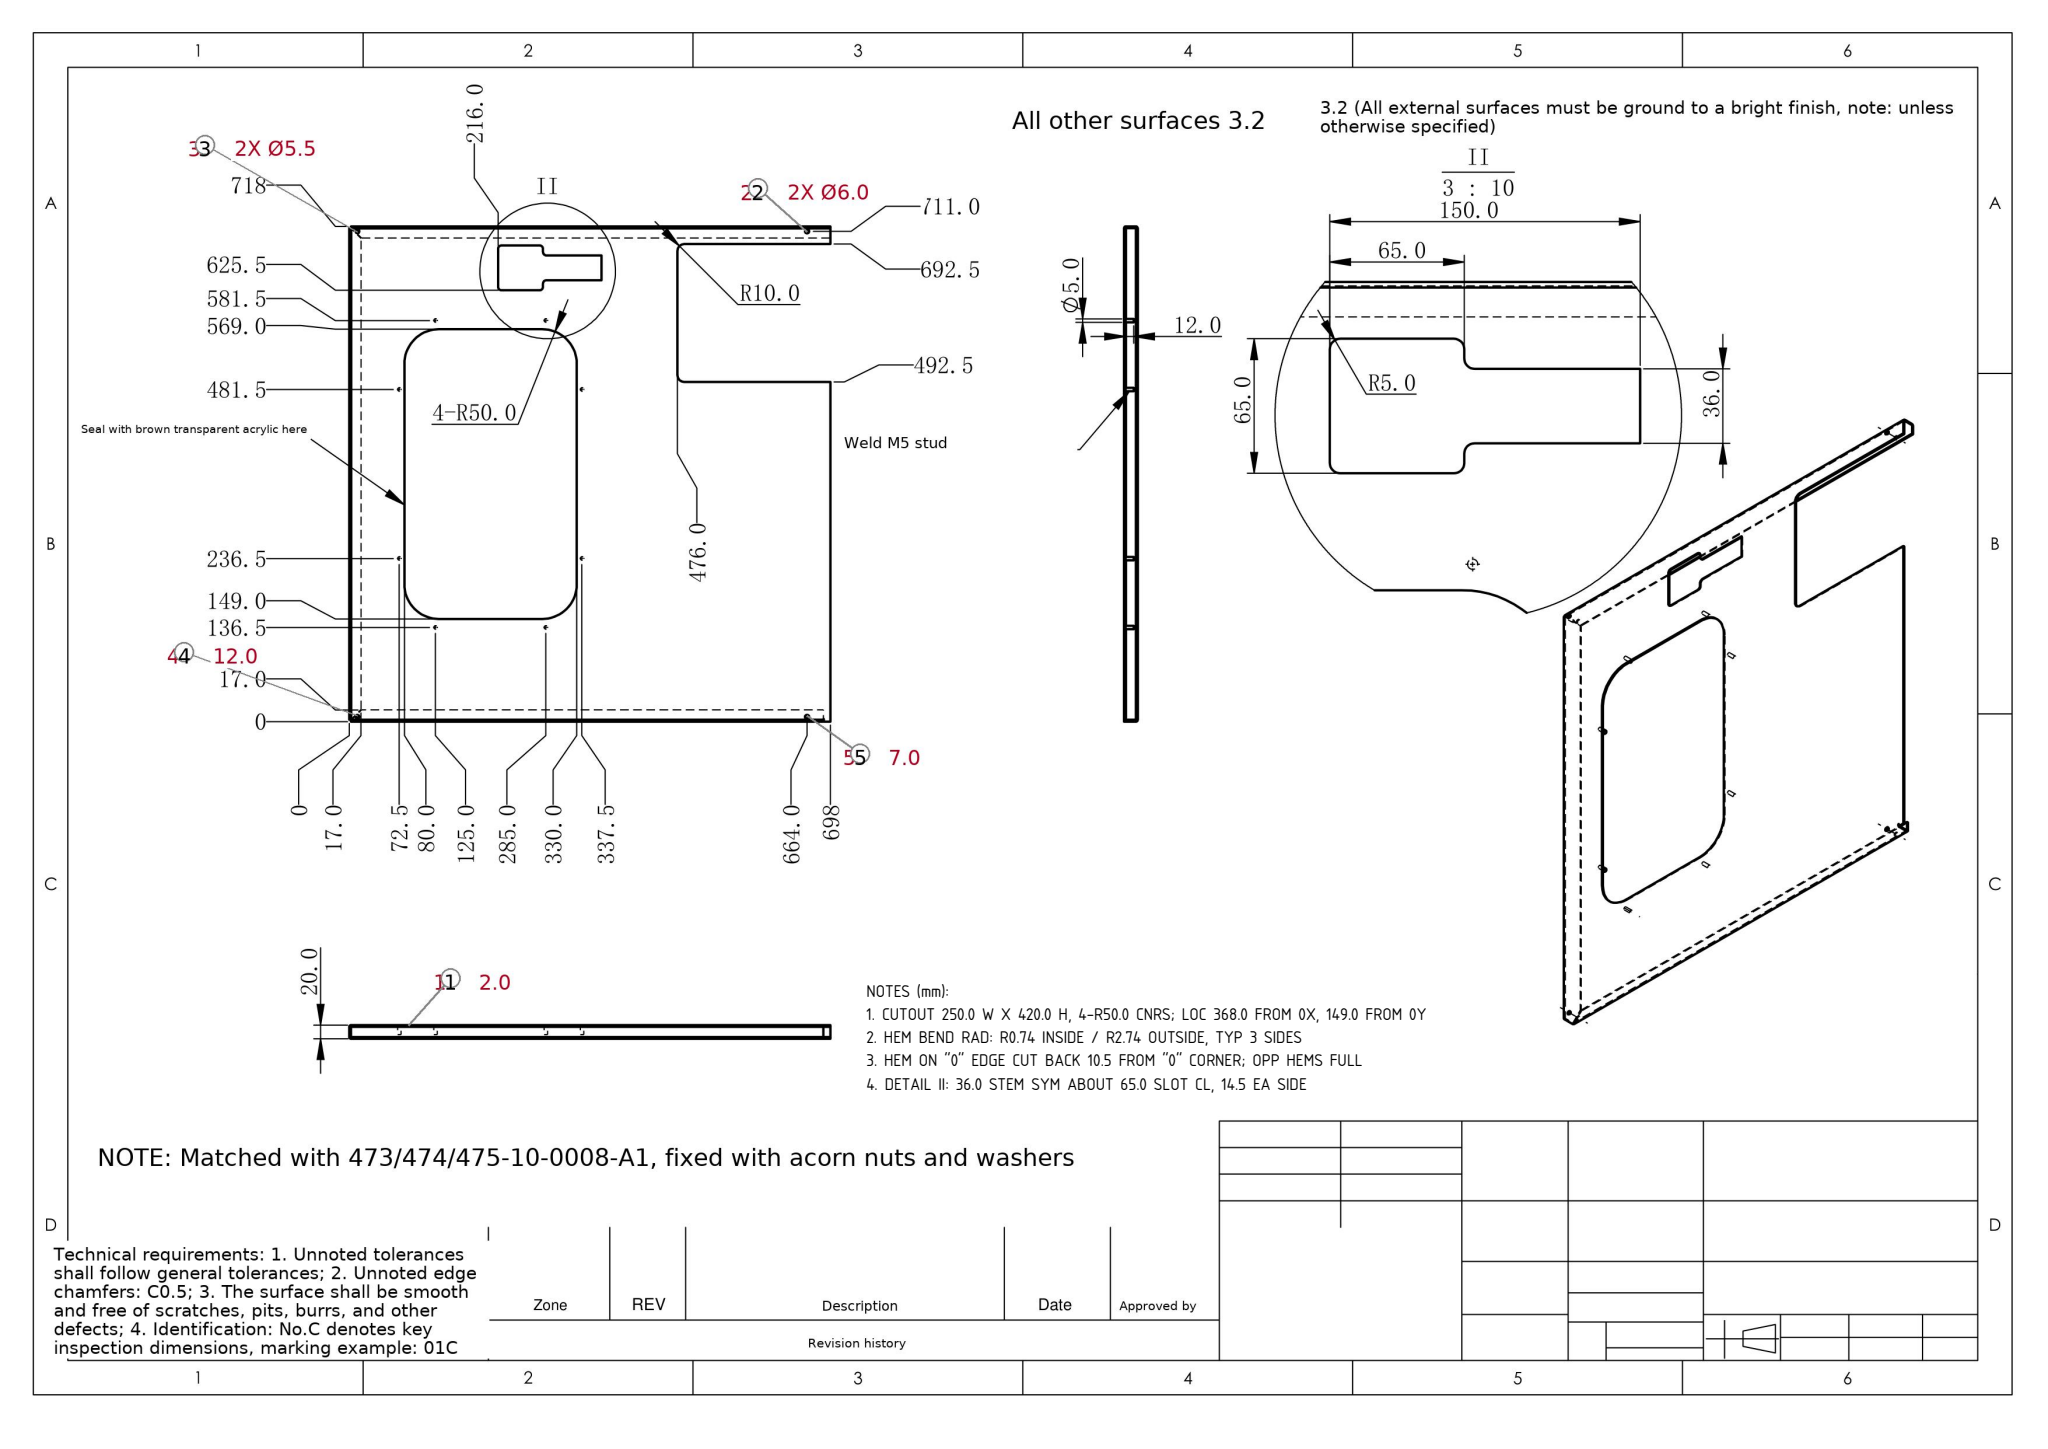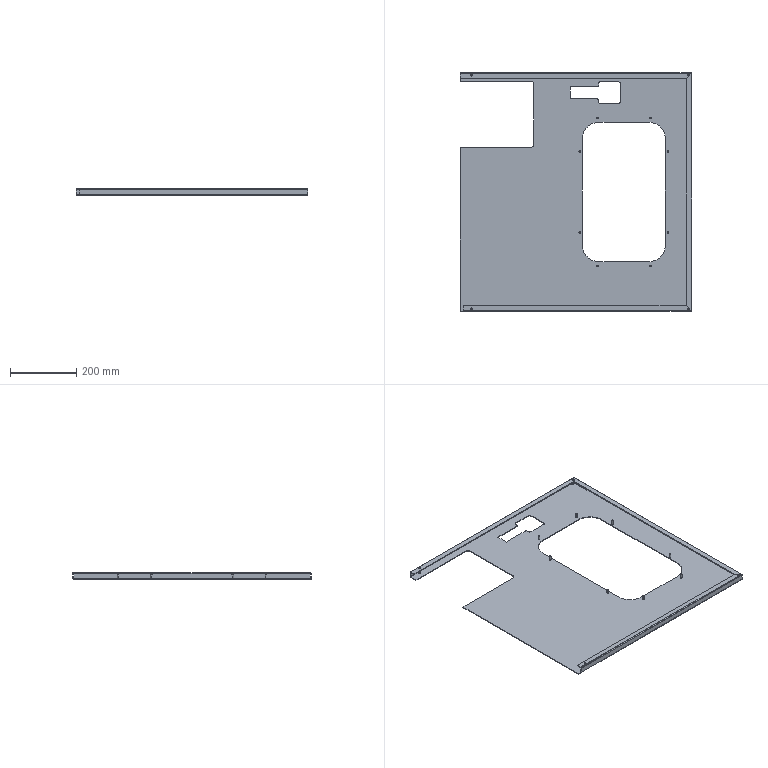Part | SolidWorks | mm | 1 solid | 126 faces | box 698 x 718 x 20 mm | volume 825760 mm3 | plane 62 | cylinder 56 | spline 8 | commonest cylinder face diameters 5 x16 6 x8 5.5 x8 5.473 x6 1.473 x6 10 x6 100 x4 20 x2
Drawing notes:
CUTOUT 250.0 W X 420.0 H, 4-R50.0 CNRS; LOC 368.0 FROM 0X, 149.0 FROM 0Y | from the solid: Four dia 100 (R50) corner cyls at x=418/568, y=199/519 -> 150+100=250 W, 320+100=420 H; cutout edges x 368-618, y 149-569
HEM BEND RAD: R0.74 INSIDE / R2.74 OUTSIDE, TYP 3 SIDES | from the solid: Hem bend cylinders dia 1.473 (R0.736) inner and dia 5.473 (R2.736) outer, axes x at y=2.76 & y=715.28 and axis y at x=695.26
HEM ON "0" EDGE CUT BACK 10.5 FROM "0" CORNER; OPP HEMS FULL | from the solid: x-axis hem at y=2.76 len 684.79 starts at plane x=10.5 (relief face x=9.5/10.5); hem at y=715.28 len 695.29 runs from x=0 to 695.29
DETAIL II: 36.0 STEM SYM ABOUT 65.0 SLOT CL, 14.5 EA SIDE | from the solid: y planes 625.52 & 690.52 (65.0 blk) vs 640.02 & 676.02 (36.0 stem); both centered at y=658.02